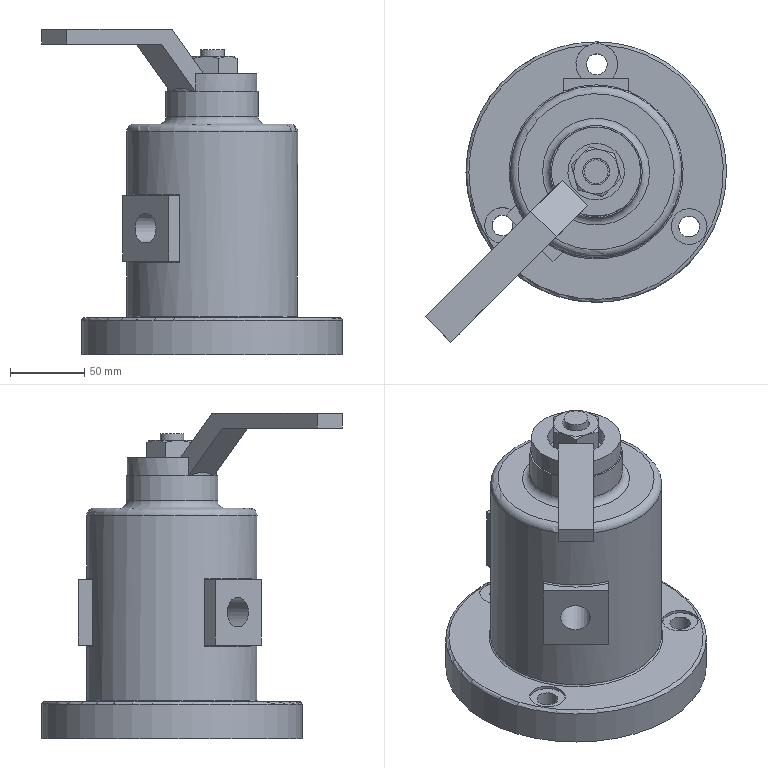Assembly | NX | mm | 7 component files | 7 solids | 104 faces | box 202.05 x 202.05 x 218.82 mm | volume 2024495 mm3 | plane 51 | cylinder 28 | cone 17 | torus 8 | commonest cylinder face diameters 18 x3 20 x3 14 x3 60 x2 4 x2 24 x2 45 x2 38 x1
Bill of materials:
unnamed part 1 | 1 |  | Plain solid short cylinder (disc). Its diameter is clearly larger than its height.
unnamed part 2 | 1 |  | Stepped cylindrical pin. A wide disc-shaped flange forms the base. A longer middle shaft rises from it, and a slightly narrower top shaft continues on the same axis.
unnamed part 3 | 1 |  | Flanged cylindrical housing. A round base flange has three equally spaced through holes. A large cylindrical body with a rounded top edge sits on it, topped by a smaller cylindrical boss with a central hole. Two rectangular pads stand out from opposite sides of the body, and at least one has a cross hole.
GB-T41-2000,M20x2.5 | 1 |  | Hexagonal prism with a central cylindrical through-bore along the hex axis and conical chamfers on both end faces, giving a shape like a hex nut.
unnamed part 4 | 1 |  | Flat strip of rectangular cross-section, bent into a Z-shaped offset (joggle). It ends in a flat ring (annular eye) lying in the lower plane.
unnamed part 5 | 1 |  | Plain solid cylinder with a height roughly equal to its diameter (slightly less).
GB93-87,(18) | 1 |  | Single Coil Spring Lock Washer, Normal Type, GB 93-87,(18)
Mates:
1. touch align | screw_plug 1 face | valve_seat 1 face
2. touch align | screw_plug 1 face | valve_seat 1 face
3. touch align | plug 1 | valve_seat 1 face
4. concentric | plug 1 | valve_seat 1 edge
5. touch align | valve_core 1 face | valve_seat 1 face
6. touch align | wrench 1 face | valve_seat 1 face
7. touch align | wrench 1 face | valve_seat 1 face
8. touch align | GB-T41-2000_M20x2_5 1 | valve_core 1 face
9. touch align | valve_core 1 face | valve_seat 1 face
10. parallel | GB-T41-2000_M20x2_5 1 | valve_seat 1 face
11. touch align | GB93-87__18 1 | GB-T41-2000_M20x2_5 1
12. touch align | GB93-87__18 1 | GB-T41-2000_M20x2_5 1
13. touch align | GB93-87__18 1 | valve_seat 1 face
14. align lock | valve_seat 1 face | valve_core 1 face
15. distance | wrench 1 face | valve_seat 1 face